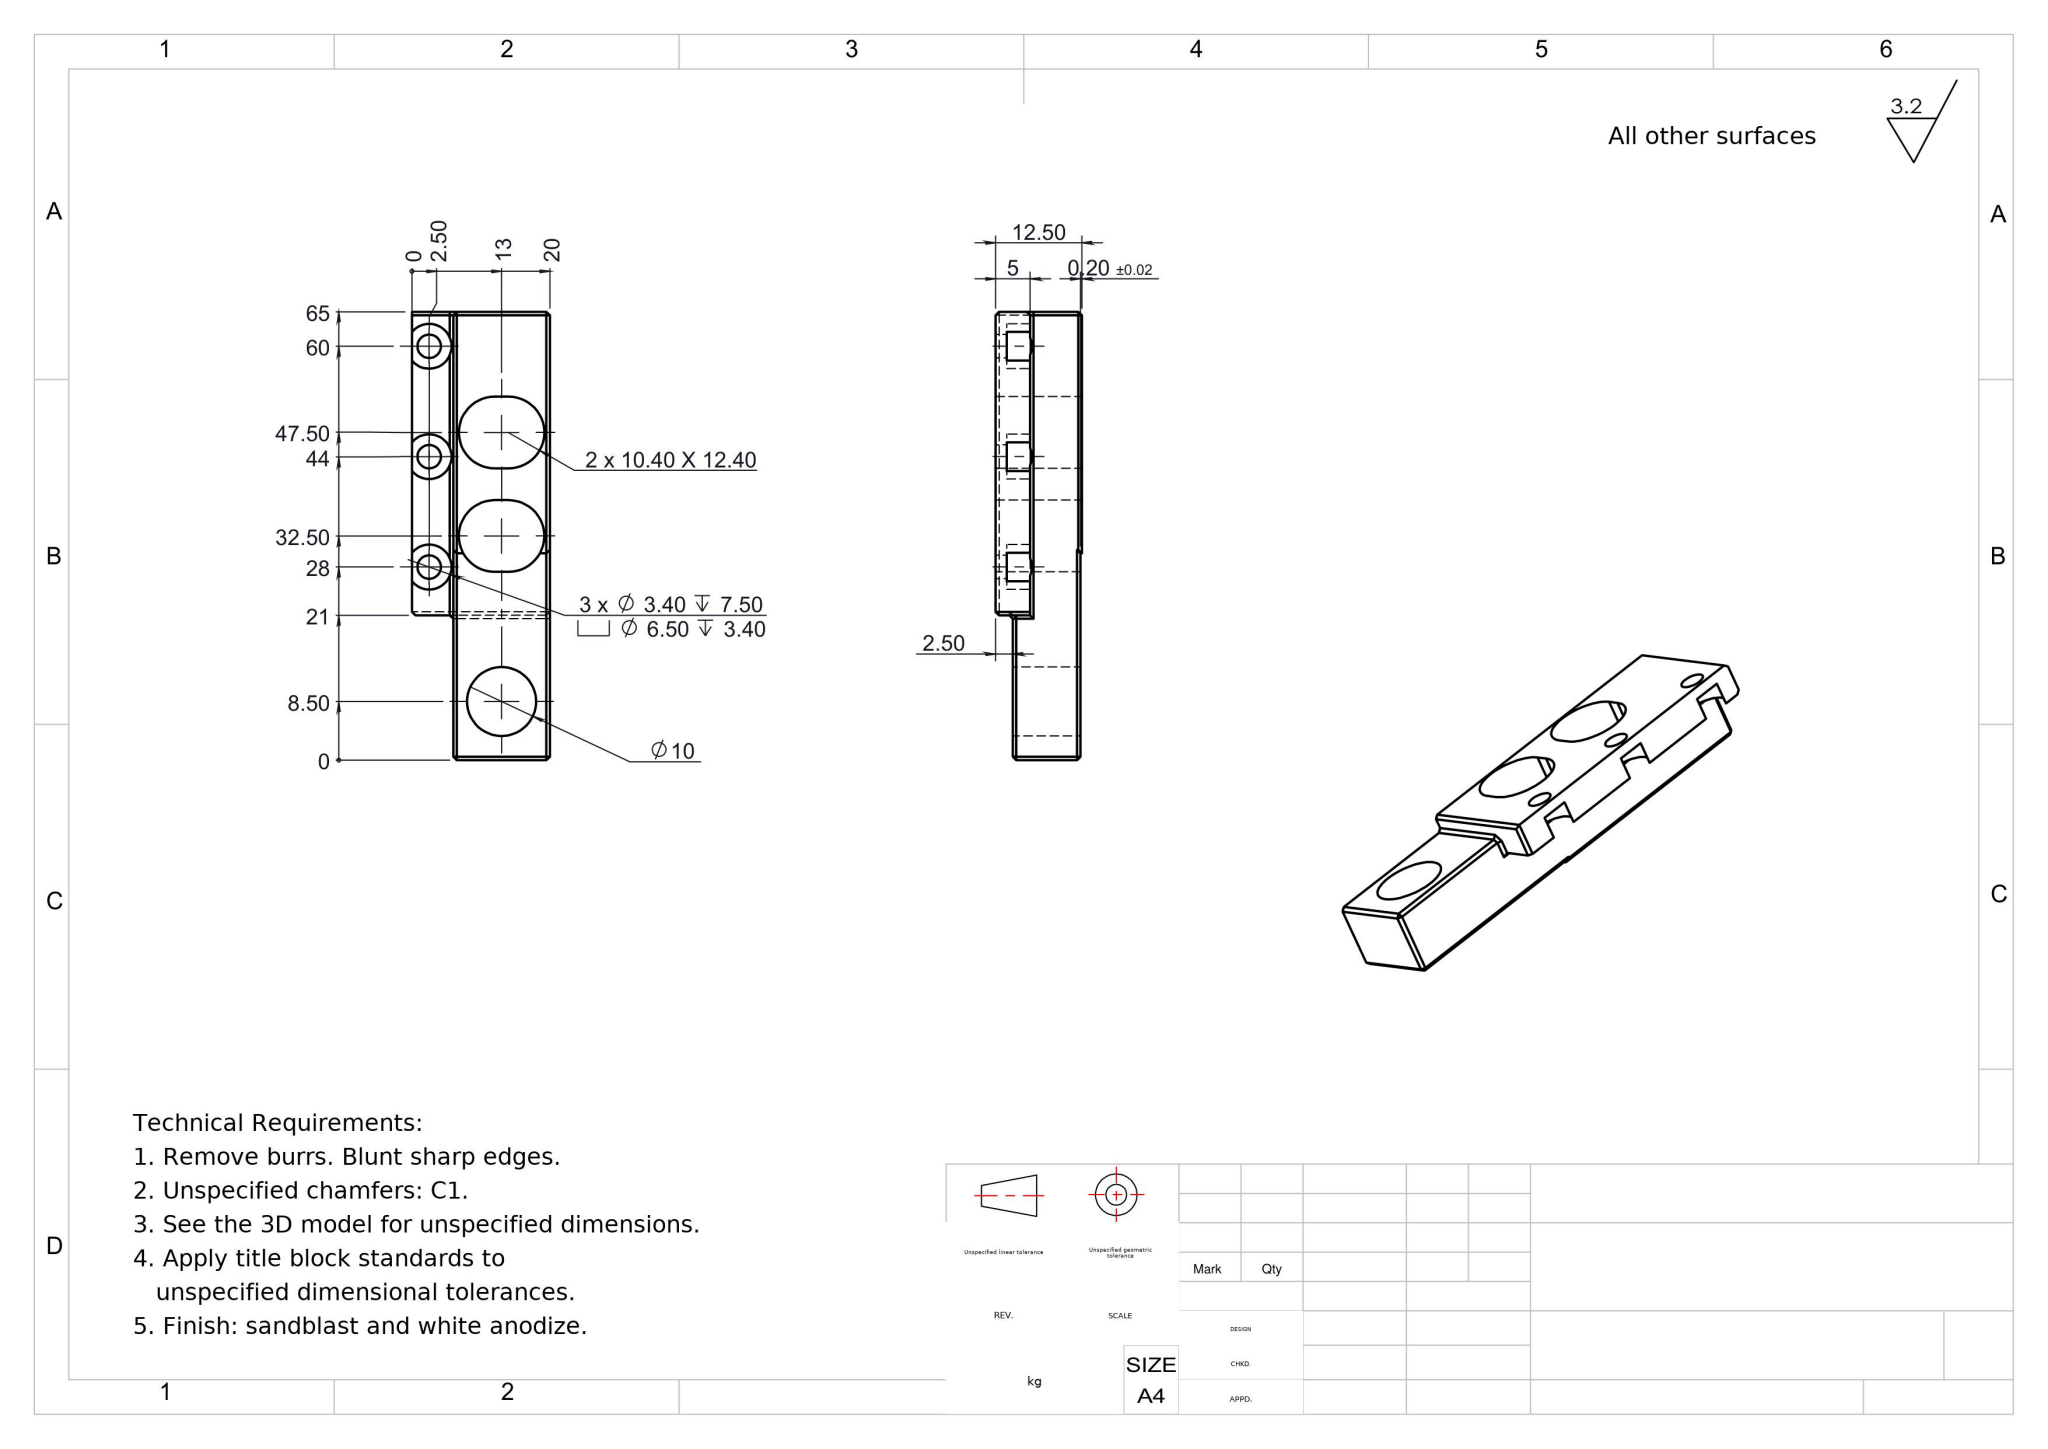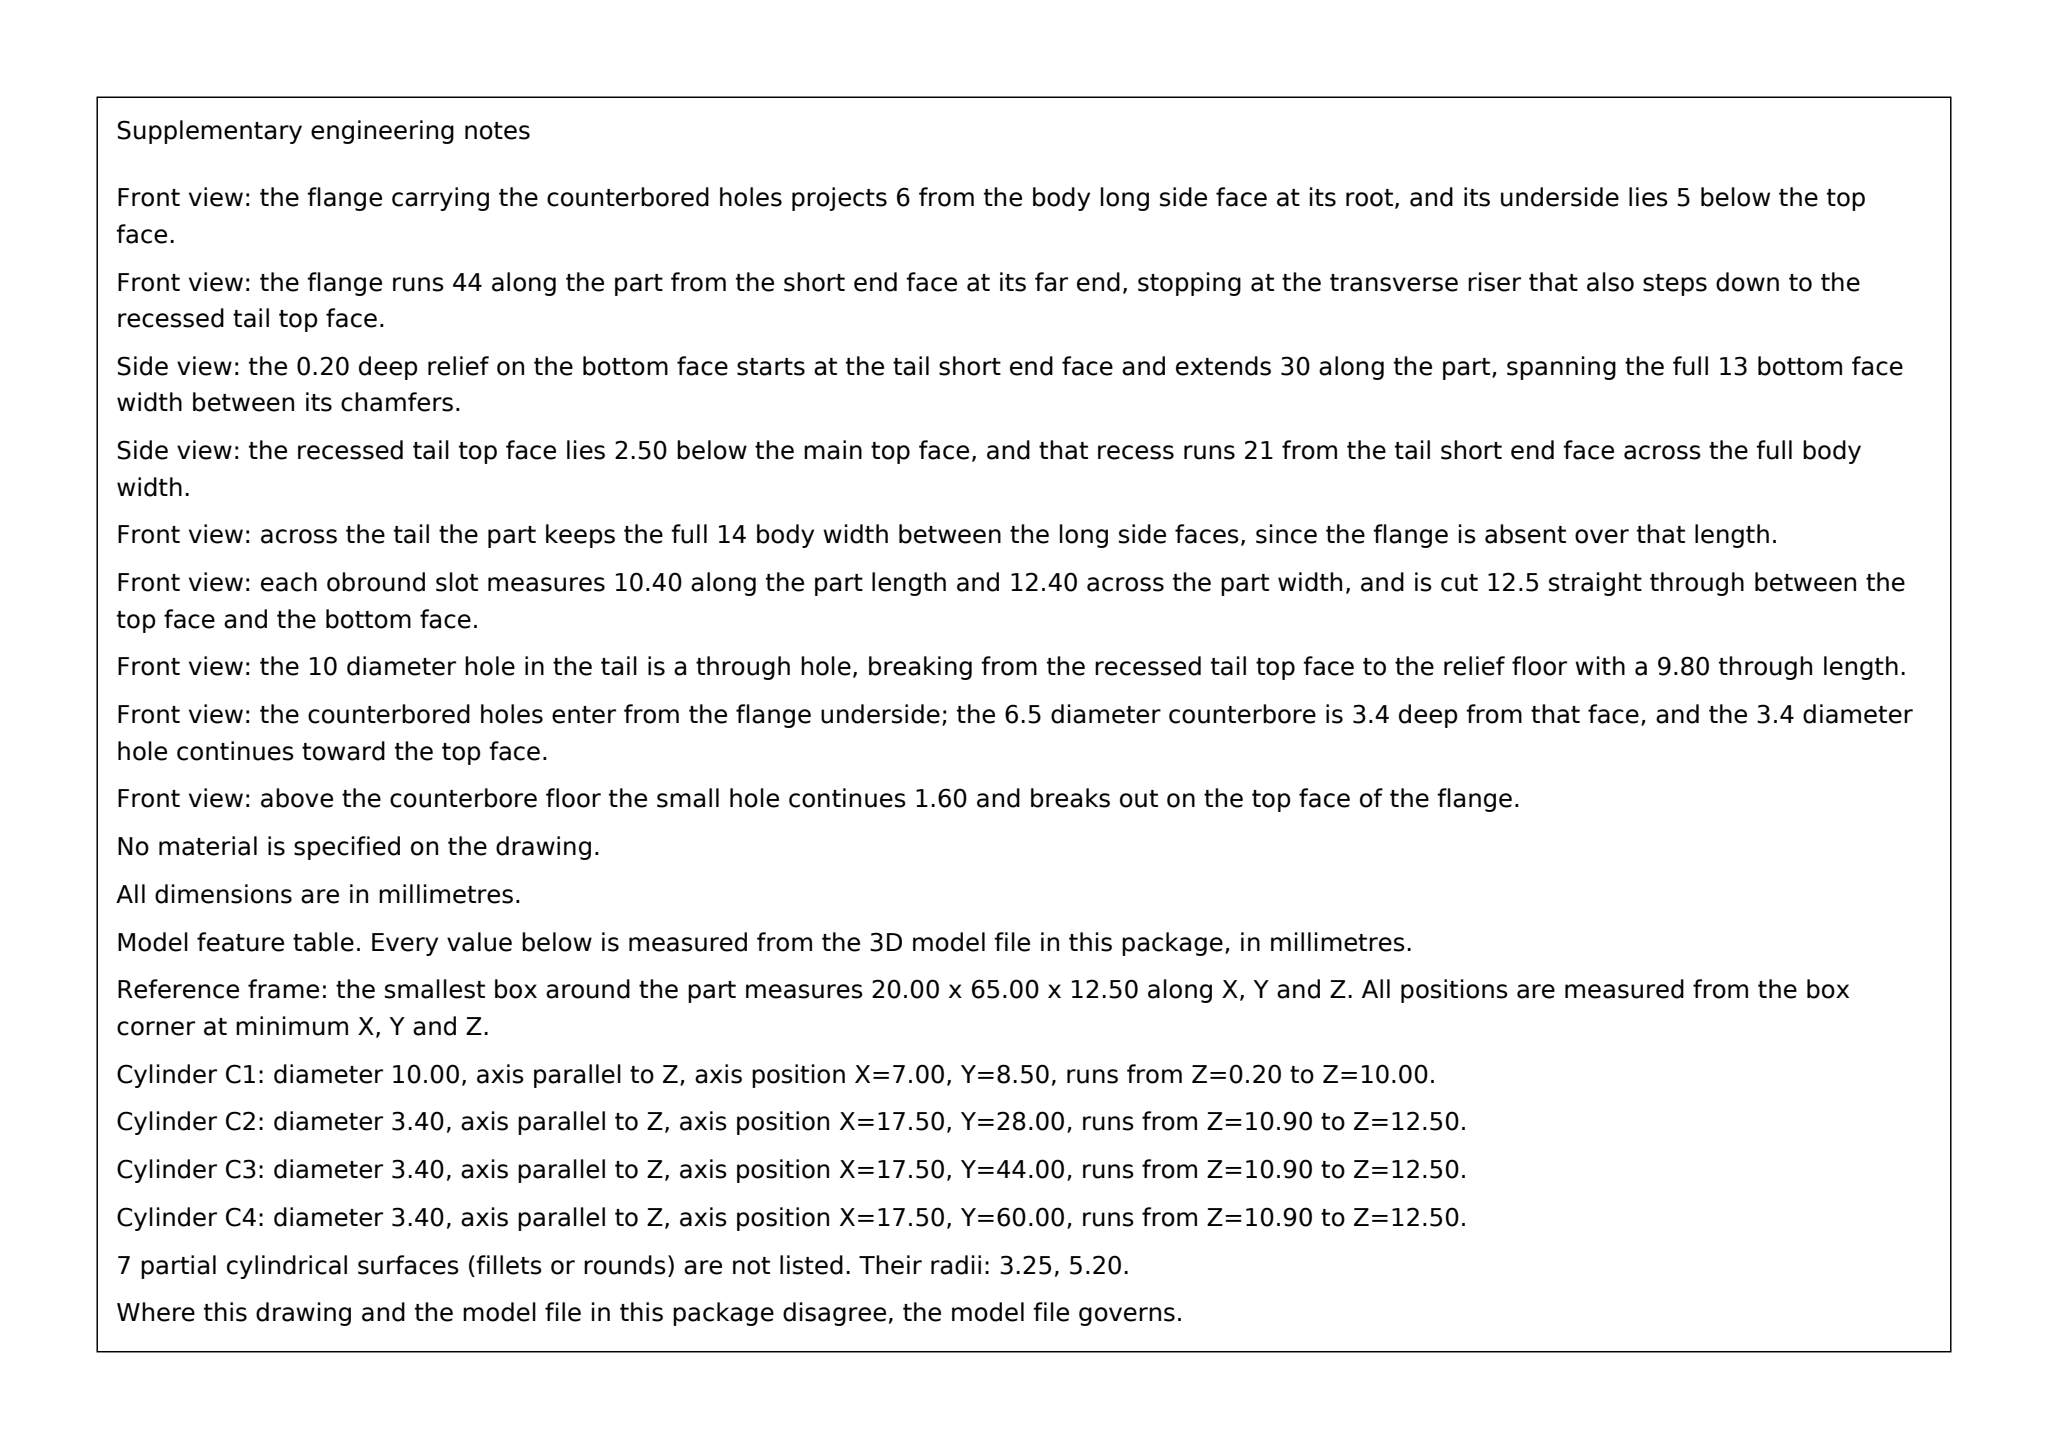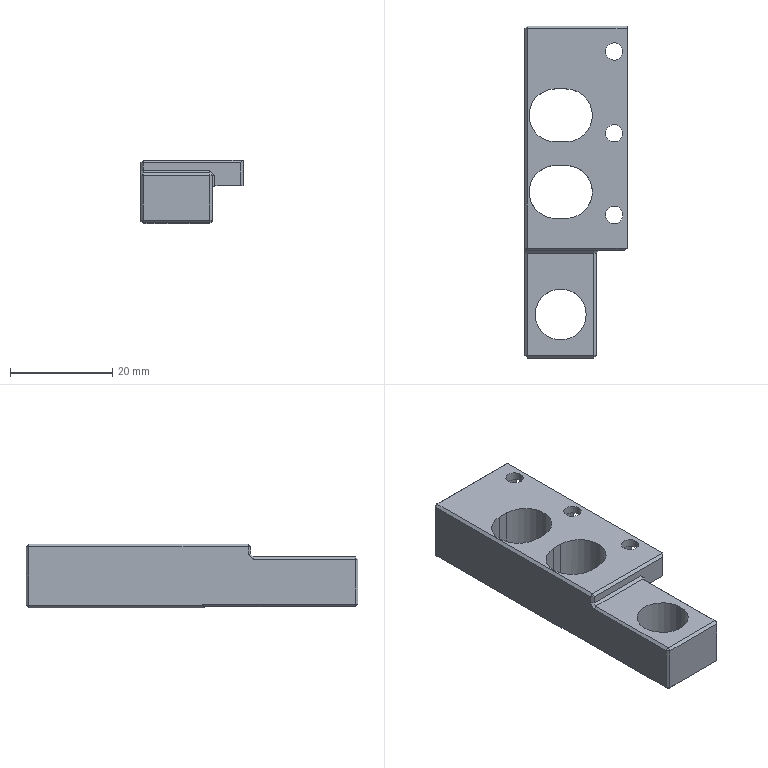Part | SolidWorks | mm | 1 solid | 78 faces | box 20 x 65 x 12.5 mm | volume 8071 mm3 | plane 58 | cylinder 20 | commonest cylinder face diameters 6.5 x6 3.4 x6 10.4 x6 10 x2
Drawing notes:
STOCK 20 X 65 X 12.50 | from the solid: bbox_xyz [20.0, 65.0, 12.5]
STEP: Y 0 TO 21, FULL 20 WIDE, 2.50 DP FROM FRONT FACE | from the solid: y plane 21.0; z plane 10.0 vs front face z=12.5 -> 2.50 step; x extent 0-20
SIDE RECESS 6 WIDE FROM 0 DATUM X 5 DP FROM FRONT FACE | from the solid: x plane 14.0 (20-14=6 from drawing 0 datum); z plane 7.5 = 12.5-5
BACK FACE RELIEF 0.20 ±0.02 OVER RECESSED AREA | from the solid: z plane 0.2 parallel to back face z=0
2X 10.40 X 12.40 OBROUND POCKET THRU (12.50) | from the solid: Ø10.4 cyls length 12.5 = full Z thickness; arc centers 2.0 apart -> 12.40 overall
Ø10 DP 9.80, FROM 0.20 RELIEF FACE TO Z=10 FACE | from the solid: Ø10 cyl length 9.8 between z planes 0.2 and 10.0
3X CBORE Ø6.50 DP 3.40 FROM STEP FACE 5 BELOW FRONT FACE | from the solid: Ø6.5 bores z 7.2->10.9 open at plane z=7.5 (step face, 5 below z=12.5 front face); 10.9-7.5=3.40 deep
Ø3.40 CONT THRU 1.60 FROM CBORE BTM, BREAKS OUT OPP FACE | from the solid: Ø3.4 holes z 10.9->12.5 = 1.60, exit at plane z=12.5
3X CBORE HOLES ON CL 2.50 FROM BACK EDGE (X=17.5 OF 20) | from the solid: cylinder axes at x=17.5 with bbox x 0-20
0.20 ±0.02 BACK FACE RELIEF: FROM 0 TO 30 (Y DATUM), FULL 13 WIDTH | from the solid: plane z=0.2 extent x[0.5,13.5] y[0.5,30.0]; plane z=0.0 y[30.0,64.5]